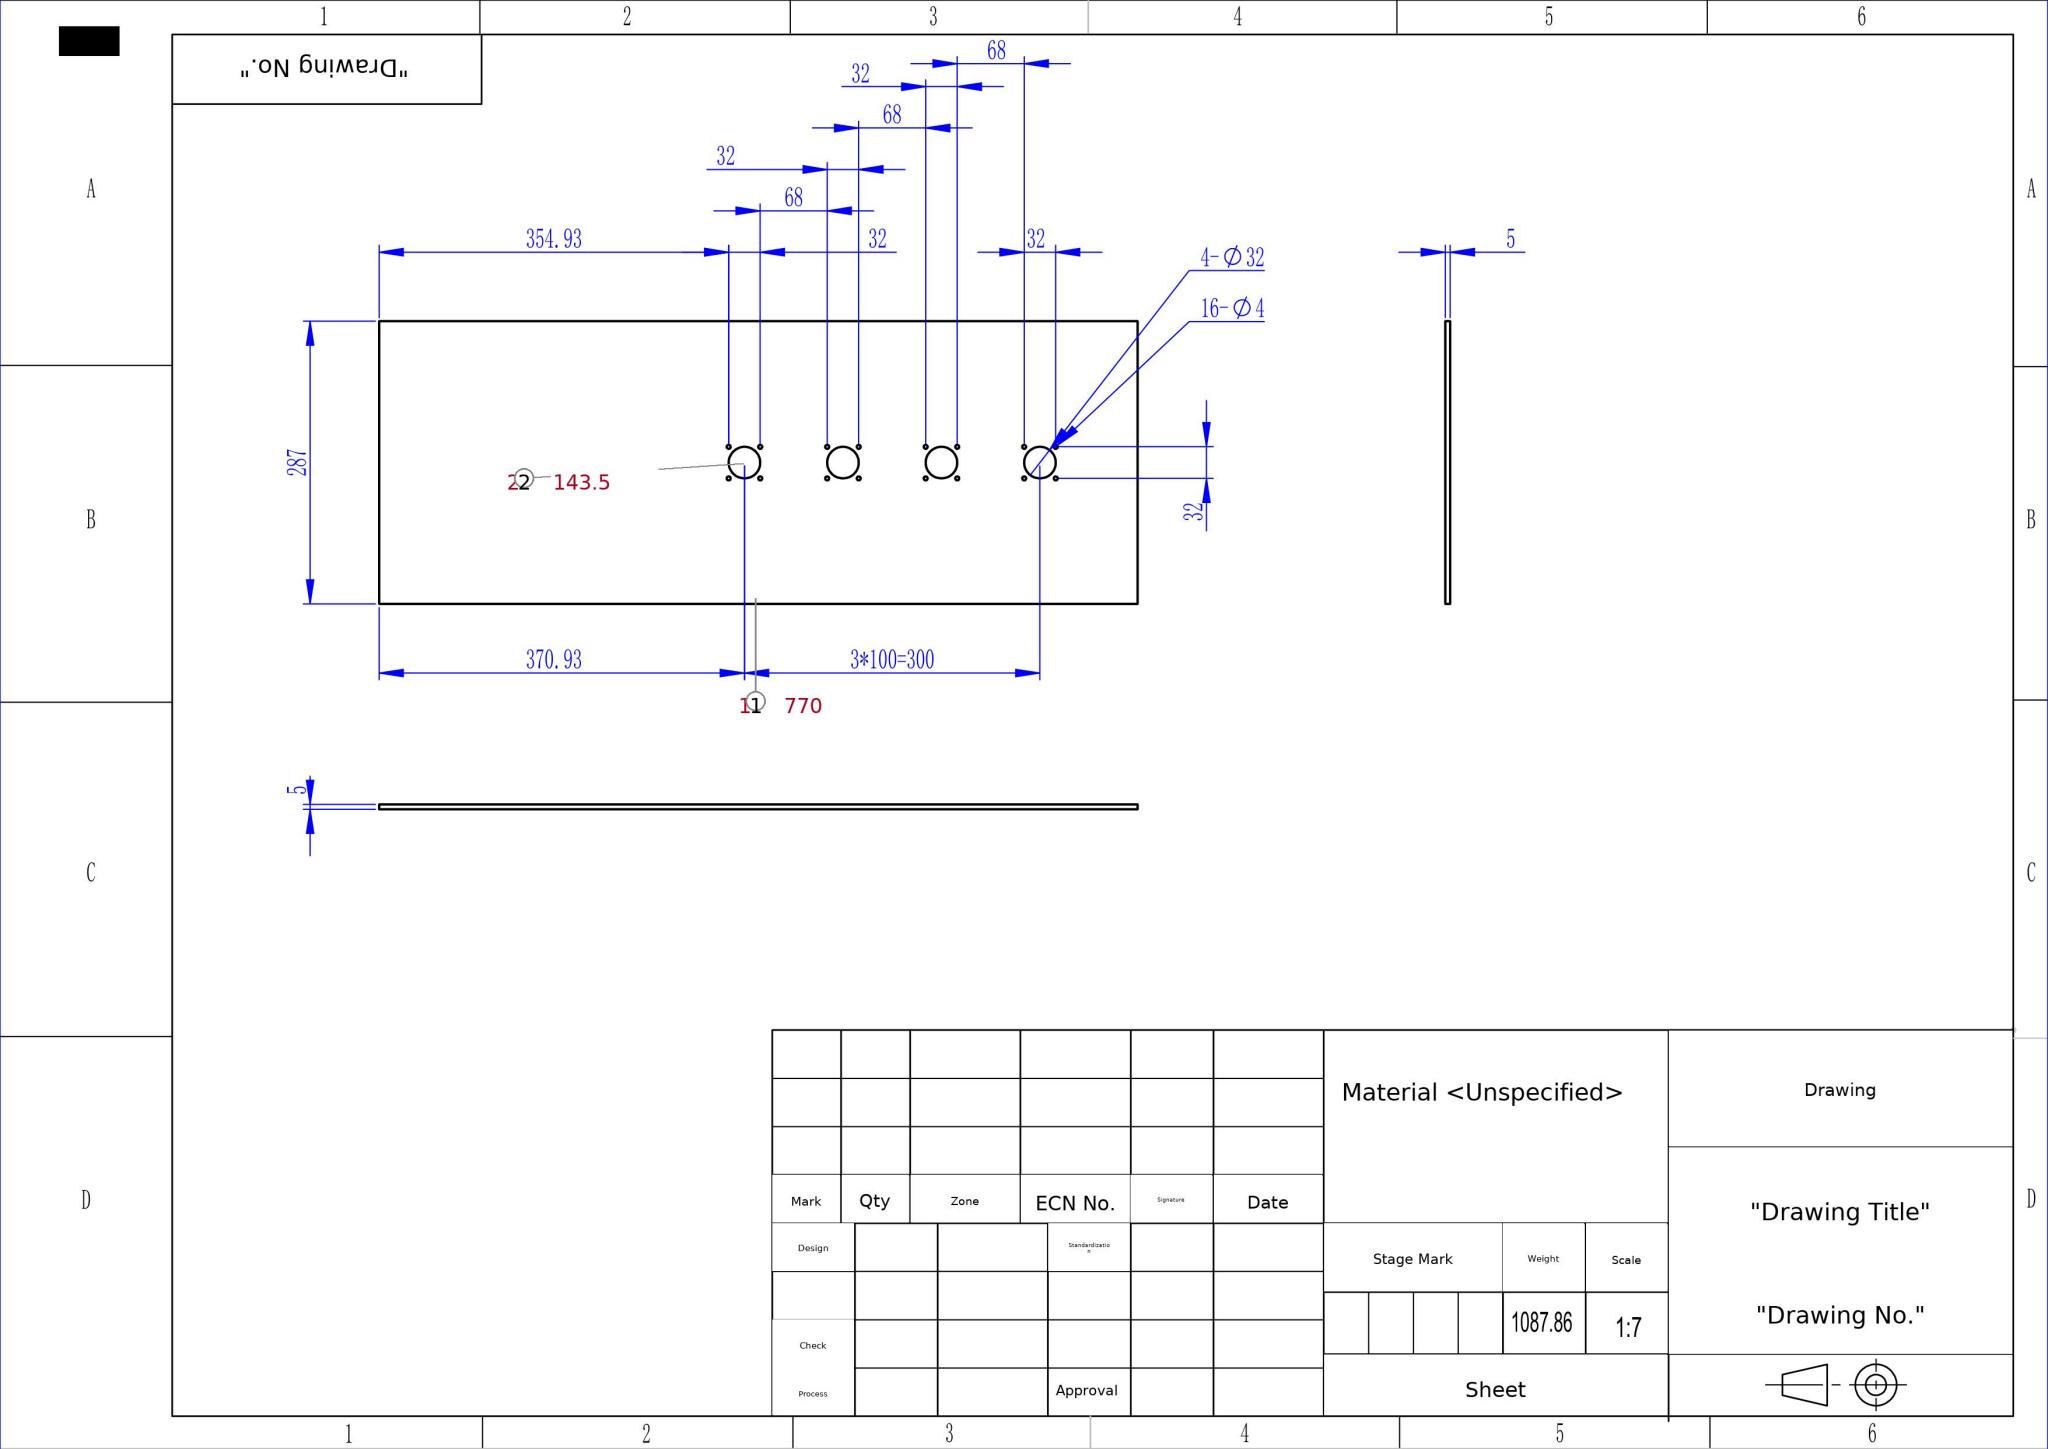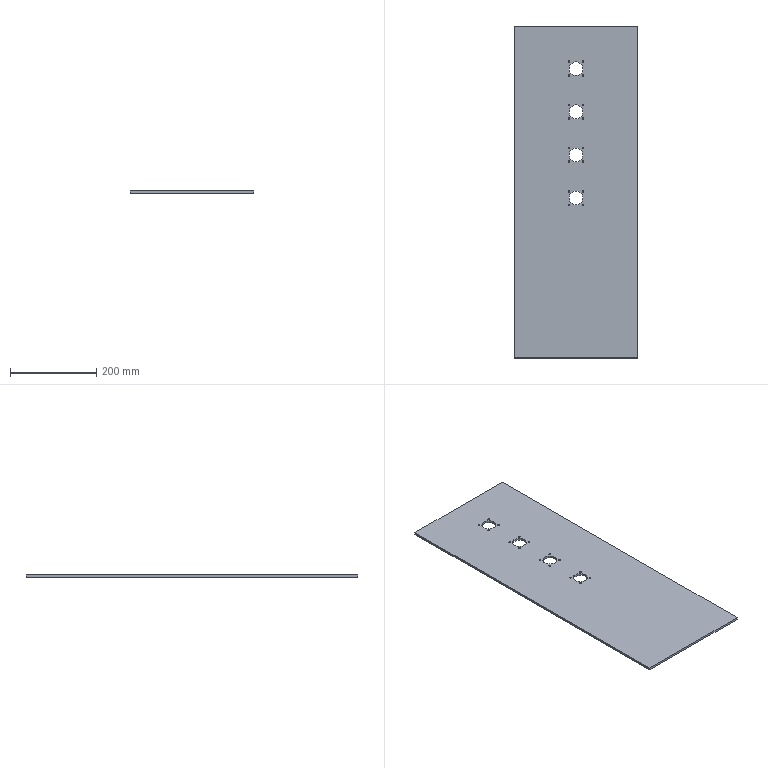Part | SolidWorks | mm | material Unspecified | 1 solid | 46 faces | box 287 x 770 x 5 mm | volume 1087860 mm3 | cylinder 40 | plane 6 | commonest cylinder face diameters 4 x32 32 x8
build123d program:
from build123d import *

# Parameters (mm, degrees)
SKETCH1_W           = 287
SKETCH1_H           = 770
SKETCH1_R           = 2
SKETCH1_R_2         = 16
BOSS_EXTRUDE1_DEPTH = 5


with BuildPart() as part:
    # Sketch1 → Boss-Extrude1 (new body)
    with BuildSketch(Plane.XY):
        Rectangle(SKETCH1_W, SKETCH1_H)
        with Locations((-16, 301.926)):
            Circle(SKETCH1_R, mode=Mode.SUBTRACT)
        with Locations((16, 301.926)):
            Circle(SKETCH1_R, mode=Mode.SUBTRACT)
        with Locations((16, 269.926)):
            Circle(SKETCH1_R, mode=Mode.SUBTRACT)
        with Locations((-16, 269.926)):
            Circle(SKETCH1_R, mode=Mode.SUBTRACT)
        with Locations((0, 285.926)):
            Circle(SKETCH1_R_2, mode=Mode.SUBTRACT)
        with Locations((-16, 201.926)):
            Circle(SKETCH1_R, mode=Mode.SUBTRACT)
        with Locations((16, 201.926)):
            Circle(SKETCH1_R, mode=Mode.SUBTRACT)
        with Locations((16, 169.926)):
            Circle(SKETCH1_R, mode=Mode.SUBTRACT)
        with Locations((-16, 169.926)):
            Circle(SKETCH1_R, mode=Mode.SUBTRACT)
        with Locations((0, 185.926)):
            Circle(SKETCH1_R_2, mode=Mode.SUBTRACT)
        with Locations((-16, 101.926)):
            Circle(SKETCH1_R, mode=Mode.SUBTRACT)
        with Locations((16, 101.926)):
            Circle(SKETCH1_R, mode=Mode.SUBTRACT)
        with Locations((16, 69.926)):
            Circle(SKETCH1_R, mode=Mode.SUBTRACT)
        with Locations((-16, 69.926)):
            Circle(SKETCH1_R, mode=Mode.SUBTRACT)
        with Locations((0, 85.926)):
            Circle(SKETCH1_R_2, mode=Mode.SUBTRACT)
        with Locations((-16, 1.926)):
            Circle(SKETCH1_R, mode=Mode.SUBTRACT)
        with Locations((16, 1.926)):
            Circle(SKETCH1_R, mode=Mode.SUBTRACT)
        with Locations((16, -30.074)):
            Circle(SKETCH1_R, mode=Mode.SUBTRACT)
        with Locations((-16, -30.074)):
            Circle(SKETCH1_R, mode=Mode.SUBTRACT)
        with Locations((0, -14.074)):
            Circle(SKETCH1_R_2, mode=Mode.SUBTRACT)
    extrude(amount=BOSS_EXTRUDE1_DEPTH)


solid = part.part